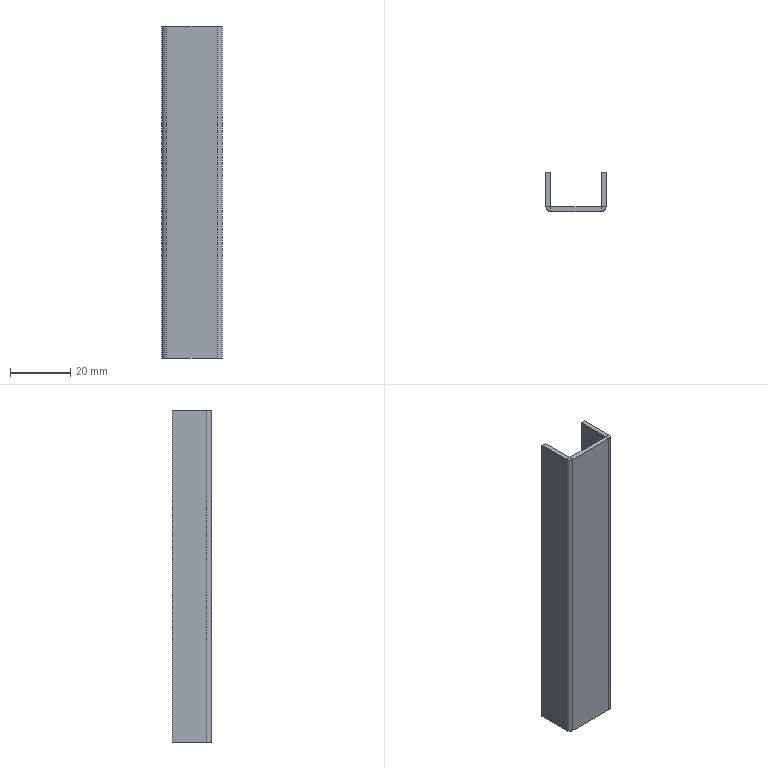Component | SolidWorks | P16BoxWeldment-1_BoxSupport-1 | 1 solid | 22 faces | box 20 x 13 x 110.6 mm | volume 7013 mm3 | plane 18 | cylinder 4 | commonest cylinder face diameters 3.2 x2 0.2 x2
STEP:
#1=COLOUR_RGB('',0.7922,0.8196,0.9333);
#2=FILL_AREA_STYLE_COLOUR('',#1);
#3=FILL_AREA_STYLE('',(#2));
#4=SURFACE_STYLE_FILL_AREA(#3);
#5=SURFACE_SIDE_STYLE('',(#4));
#6=SURFACE_STYLE_USAGE(.BOTH.,#5);
#7=PRESENTATION_STYLE_ASSIGNMENT((#6));
#8=CARTESIAN_POINT('',(-3.126,0.3402,2.409));
#9=VERTEX_POINT('',#8);
#10=CARTESIAN_POINT('',(-3.067,0.3402,2.409));
#11=VERTEX_POINT('',#10);
#12=CARTESIAN_POINT('',(-3.126,0.3402,2.409));
#13=DIRECTION('',(1.,0.,0.));
#14=VECTOR('',#13,39.37);
#15=LINE('',#12,#14);
#16=EDGE_CURVE('',#9,#11,#15,.T.);
#17=ORIENTED_EDGE('',*,*,#16,.F.);
#18=CARTESIAN_POINT('',(-3.063,0.2772,2.409));
#19=VERTEX_POINT('',#18);
#20=CARTESIAN_POINT('',(-3.063,0.3402,2.409));
#21=DIRECTION('',(0.,0.,-1.));
#22=DIRECTION('',(-1.,0.,0.));
#23=AXIS2_PLACEMENT_3D('',#20,#21,#22);
#24=CIRCLE('',#23,0.06299);
#25=EDGE_CURVE('',#19,#9,#24,.T.);
#26=ORIENTED_EDGE('',*,*,#25,.F.);
#27=CARTESIAN_POINT('',(-3.063,0.3363,2.409));
#28=VERTEX_POINT('',#27);
#29=CARTESIAN_POINT('',(-3.063,0.3363,2.409));
#30=DIRECTION('',(0.,-1.,0.));
#31=VECTOR('',#30,39.37);
#32=LINE('',#29,#31);
#33=EDGE_CURVE('',#28,#19,#32,.T.);
#34=ORIENTED_EDGE('',*,*,#33,.F.);
#35=CARTESIAN_POINT('',(-3.063,0.3402,2.409));
#36=DIRECTION('',(0.,0.,-1.));
#37=DIRECTION('',(1.,0.,0.));
#38=AXIS2_PLACEMENT_3D('',#35,#36,#37);
#39=CIRCLE('',#38,0.003937);
#40=EDGE_CURVE('',#28,#11,#39,.T.);
#41=ORIENTED_EDGE('',*,*,#40,.T.);
#42=EDGE_LOOP('',(#17,#26,#34,#41));
#43=FACE_OUTER_BOUND('',#42,.T.);
#44=CARTESIAN_POINT('',(-3.126,0.3402,2.409));
#45=DIRECTION('',(0.,0.,1.));
#46=DIRECTION('',(1.,0.,0.));
#47=AXIS2_PLACEMENT_3D('',#44,#45,#46);
#48=PLANE('',#47);
#49=ADVANCED_FACE('',(#43),#48,.T.);
#50=CARTESIAN_POINT('',(-3.126,0.7891,2.409));
#51=VERTEX_POINT('',#50);
#52=CARTESIAN_POINT('',(-3.126,0.7891,2.409));
#53=DIRECTION('',(-0.,1.,0.));
#54=VECTOR('',#53,39.37);
#55=LINE('',#52,#54);
#56=EDGE_CURVE('',#9,#51,#55,.T.);
#57=ORIENTED_EDGE('',*,*,#56,.F.);
#58=ORIENTED_EDGE('',*,*,#16,.T.);
#59=CARTESIAN_POINT('',(-3.067,0.7891,2.409));
#60=VERTEX_POINT('',#59);
#61=CARTESIAN_POINT('',(-3.067,0.7891,2.409));
#62=DIRECTION('',(-0.,1.,0.));
#63=VECTOR('',#62,39.37);
#64=LINE('',#61,#63);
#65=EDGE_CURVE('',#11,#60,#64,.T.);
#66=ORIENTED_EDGE('',*,*,#65,.T.);
#67=CARTESIAN_POINT('',(-3.126,0.7891,2.409));
#68=DIRECTION('',(1.,0.,0.));
#69=VECTOR('',#68,39.37);
#70=LINE('',#67,#69);
#71=EDGE_CURVE('',#51,#60,#70,.T.);
#72=ORIENTED_EDGE('',*,*,#71,.F.);
#73=EDGE_LOOP('',(#57,#58,#66,#72));
#74=FACE_OUTER_BOUND('',#73,.T.);
#75=CARTESIAN_POINT('',(-3.063,0.3363,2.409));
#76=DIRECTION('',(0.,0.,1.));
#77=DIRECTION('',(1.,0.,0.));
#78=AXIS2_PLACEMENT_3D('',#75,#76,#77);
#79=PLANE('',#78);
#80=ADVANCED_FACE('',(#74),#79,.T.);
#81=CARTESIAN_POINT('',(-3.063,0.2772,-1.945));
#82=VERTEX_POINT('',#81);
#83=CARTESIAN_POINT('',(-3.063,0.3363,-1.945));
#84=VERTEX_POINT('',#83);
#85=CARTESIAN_POINT('',(-3.063,0.2772,-1.945));
#86=DIRECTION('',(0.,1.,0.));
#87=VECTOR('',#86,39.37);
#88=LINE('',#85,#87);
#89=EDGE_CURVE('',#82,#84,#88,.T.);
#90=ORIENTED_EDGE('',*,*,#89,.F.);
#91=CARTESIAN_POINT('',(-3.126,0.3402,-1.945));
#92=VERTEX_POINT('',#91);
#93=CARTESIAN_POINT('',(-3.063,0.3402,-1.945));
#94=DIRECTION('',(0.,0.,-1.));
#95=DIRECTION('',(-1.,0.,0.));
#96=AXIS2_PLACEMENT_3D('',#93,#94,#95);
#97=CIRCLE('',#96,0.06299);
#98=EDGE_CURVE('',#82,#92,#97,.T.);
#99=ORIENTED_EDGE('',*,*,#98,.T.);
#100=CARTESIAN_POINT('',(-3.067,0.3402,-1.945));
#101=VERTEX_POINT('',#100);
#102=CARTESIAN_POINT('',(-3.067,0.3402,-1.945));
#103=DIRECTION('',(-1.,0.,0.));
#104=VECTOR('',#103,39.37);
#105=LINE('',#102,#104);
#106=EDGE_CURVE('',#101,#92,#105,.T.);
#107=ORIENTED_EDGE('',*,*,#106,.F.);
#108=CARTESIAN_POINT('',(-3.063,0.3402,-1.945));
#109=DIRECTION('',(0.,0.,-1.));
#110=DIRECTION('',(1.,0.,0.));
#111=AXIS2_PLACEMENT_3D('',#108,#109,#110);
#112=CIRCLE('',#111,0.003937);
#113=EDGE_CURVE('',#84,#101,#112,.T.);
#114=ORIENTED_EDGE('',*,*,#113,.F.);
#115=EDGE_LOOP('',(#90,#99,#107,#114));
#116=FACE_OUTER_BOUND('',#115,.T.);
#117=CARTESIAN_POINT('',(-3.063,0.2772,-1.945));
#118=DIRECTION('',(0.,0.,-1.));
#119=DIRECTION('',(-1.,0.,0.));
#120=AXIS2_PLACEMENT_3D('',#117,#118,#119);
#121=PLANE('',#120);
#122=ADVANCED_FACE('',(#116),#121,.T.);
#123=CARTESIAN_POINT('',(-2.401,0.2772,-1.945));
#124=VERTEX_POINT('',#123);
#125=CARTESIAN_POINT('',(-3.126,0.2772,-1.945));
#126=DIRECTION('',(-1.,-0.,0.));
#127=VECTOR('',#126,39.37);
#128=LINE('',#125,#127);
#129=EDGE_CURVE('',#124,#82,#128,.T.);
#130=ORIENTED_EDGE('',*,*,#129,.T.);
#131=ORIENTED_EDGE('',*,*,#89,.T.);
#132=CARTESIAN_POINT('',(-2.401,0.3363,-1.945));
#133=VERTEX_POINT('',#132);
#134=CARTESIAN_POINT('',(-3.126,0.3363,-1.945));
#135=DIRECTION('',(-1.,-0.,0.));
#136=VECTOR('',#135,39.37);
#137=LINE('',#134,#136);
#138=EDGE_CURVE('',#133,#84,#137,.T.);
#139=ORIENTED_EDGE('',*,*,#138,.F.);
#140=CARTESIAN_POINT('',(-2.401,0.3363,-1.945));
#141=DIRECTION('',(0.,-1.,0.));
#142=VECTOR('',#141,39.37);
#143=LINE('',#140,#142);
#144=EDGE_CURVE('',#133,#124,#143,.T.);
#145=ORIENTED_EDGE('',*,*,#144,.T.);
#146=EDGE_LOOP('',(#130,#131,#139,#145));
#147=FACE_OUTER_BOUND('',#146,.T.);
#148=CARTESIAN_POINT('',(-3.067,0.3402,-1.945));
#149=DIRECTION('',(0.,0.,-1.));
#150=DIRECTION('',(-1.,0.,0.));
#151=AXIS2_PLACEMENT_3D('',#148,#149,#150);
#152=PLANE('',#151);
#153=ADVANCED_FACE('',(#147),#152,.T.);
#154=CARTESIAN_POINT('',(-2.401,0.2772,2.409));
#155=VERTEX_POINT('',#154);
#156=CARTESIAN_POINT('',(-2.401,0.3363,2.409));
#157=VERTEX_POINT('',#156);
#158=CARTESIAN_POINT('',(-2.401,0.2772,2.409));
#159=DIRECTION('',(0.,1.,0.));
#160=VECTOR('',#159,39.37);
#161=LINE('',#158,#160);
#162=EDGE_CURVE('',#155,#157,#161,.T.);
#163=ORIENTED_EDGE('',*,*,#162,.F.);
#164=CARTESIAN_POINT('',(-2.338,0.3402,2.409));
#165=VERTEX_POINT('',#164);
#166=CARTESIAN_POINT('',(-2.401,0.3402,2.409));
#167=DIRECTION('',(0.,0.,-1.));
#168=DIRECTION('',(-1.,0.,0.));
#169=AXIS2_PLACEMENT_3D('',#166,#167,#168);
#170=CIRCLE('',#169,0.06299);
#171=EDGE_CURVE('',#165,#155,#170,.T.);
#172=ORIENTED_EDGE('',*,*,#171,.F.);
#173=CARTESIAN_POINT('',(-2.397,0.3402,2.409));
#174=VERTEX_POINT('',#173);
#175=CARTESIAN_POINT('',(-2.397,0.3402,2.409));
#176=DIRECTION('',(1.,0.,0.));
#177=VECTOR('',#176,39.37);
#178=LINE('',#175,#177);
#179=EDGE_CURVE('',#174,#165,#178,.T.);
#180=ORIENTED_EDGE('',*,*,#179,.F.);
#181=CARTESIAN_POINT('',(-2.401,0.3402,2.409));
#182=DIRECTION('',(0.,0.,-1.));
#183=DIRECTION('',(1.,0.,0.));
#184=AXIS2_PLACEMENT_3D('',#181,#182,#183);
#185=CIRCLE('',#184,0.003937);
#186=EDGE_CURVE('',#174,#157,#185,.T.);
#187=ORIENTED_EDGE('',*,*,#186,.T.);
#188=EDGE_LOOP('',(#163,#172,#180,#187));
#189=FACE_OUTER_BOUND('',#188,.T.);
#190=CARTESIAN_POINT('',(-2.401,0.2772,2.409));
#191=DIRECTION('',(0.,0.,1.));
#192=DIRECTION('',(1.,0.,0.));
#193=AXIS2_PLACEMENT_3D('',#190,#191,#192);
#194=PLANE('',#193);
#195=ADVANCED_FACE('',(#189),#194,.T.);
#196=CARTESIAN_POINT('',(-3.126,0.2772,2.409));
#197=DIRECTION('',(-1.,-0.,0.));
#198=VECTOR('',#197,39.37);
#199=LINE('',#196,#198);
#200=EDGE_CURVE('',#155,#19,#199,.T.);
#201=ORIENTED_EDGE('',*,*,#200,.F.);
#202=ORIENTED_EDGE('',*,*,#162,.T.);
#203=CARTESIAN_POINT('',(-3.126,0.3363,2.409));
#204=DIRECTION('',(-1.,-0.,0.));
#205=VECTOR('',#204,39.37);
#206=LINE('',#203,#205);
#207=EDGE_CURVE('',#157,#28,#206,.T.);
#208=ORIENTED_EDGE('',*,*,#207,.T.);
#209=ORIENTED_EDGE('',*,*,#33,.T.);
#210=EDGE_LOOP('',(#201,#202,#208,#209));
#211=FACE_OUTER_BOUND('',#210,.T.);
#212=CARTESIAN_POINT('',(-2.397,0.3402,2.409));
#213=DIRECTION('',(0.,0.,1.));
#214=DIRECTION('',(1.,0.,0.));
#215=AXIS2_PLACEMENT_3D('',#212,#213,#214);
#216=PLANE('',#215);
#217=ADVANCED_FACE('',(#211),#216,.T.);
#218=CARTESIAN_POINT('',(-2.338,0.3402,-1.945));
#219=VERTEX_POINT('',#218);
#220=CARTESIAN_POINT('',(-2.397,0.3402,-1.945));
#221=VERTEX_POINT('',#220);
#222=CARTESIAN_POINT('',(-2.338,0.3402,-1.945));
#223=DIRECTION('',(-1.,-0.,0.));
#224=VECTOR('',#223,39.37);
#225=LINE('',#222,#224);
#226=EDGE_CURVE('',#219,#221,#225,.T.);
#227=ORIENTED_EDGE('',*,*,#226,.F.);
#228=CARTESIAN_POINT('',(-2.401,0.3402,-1.945));
#229=DIRECTION('',(0.,0.,-1.));
#230=DIRECTION('',(-1.,0.,0.));
#231=AXIS2_PLACEMENT_3D('',#228,#229,#230);
#232=CIRCLE('',#231,0.06299);
#233=EDGE_CURVE('',#219,#124,#232,.T.);
#234=ORIENTED_EDGE('',*,*,#233,.T.);
#235=ORIENTED_EDGE('',*,*,#144,.F.);
#236=CARTESIAN_POINT('',(-2.401,0.3402,-1.945));
#237=DIRECTION('',(0.,0.,-1.));
#238=DIRECTION('',(1.,0.,0.));
#239=AXIS2_PLACEMENT_3D('',#236,#237,#238);
#240=CIRCLE('',#239,0.003937);
#241=EDGE_CURVE('',#221,#133,#240,.T.);
#242=ORIENTED_EDGE('',*,*,#241,.F.);
#243=EDGE_LOOP('',(#227,#234,#235,#242));
#244=FACE_OUTER_BOUND('',#243,.T.);
#245=CARTESIAN_POINT('',(-2.338,0.3402,-1.945));
#246=DIRECTION('',(0.,0.,-1.));
#247=DIRECTION('',(-1.,0.,0.));
#248=AXIS2_PLACEMENT_3D('',#245,#246,#247);
#249=PLANE('',#248);
#250=ADVANCED_FACE('',(#244),#249,.T.);
#251=CARTESIAN_POINT('',(-2.338,0.7891,-1.945));
#252=VERTEX_POINT('',#251);
#253=CARTESIAN_POINT('',(-2.338,0.7891,-1.945));
#254=DIRECTION('',(0.,-1.,0.));
#255=VECTOR('',#254,39.37);
#256=LINE('',#253,#255);
#257=EDGE_CURVE('',#252,#219,#256,.T.);
#258=ORIENTED_EDGE('',*,*,#257,.T.);
#259=ORIENTED_EDGE('',*,*,#226,.T.);
#260=CARTESIAN_POINT('',(-2.397,0.7891,-1.945));
#261=VERTEX_POINT('',#260);
#262=CARTESIAN_POINT('',(-2.397,0.7891,-1.945));
#263=DIRECTION('',(0.,-1.,0.));
#264=VECTOR('',#263,39.37);
#265=LINE('',#262,#264);
#266=EDGE_CURVE('',#261,#221,#265,.T.);
#267=ORIENTED_EDGE('',*,*,#266,.F.);
#268=CARTESIAN_POINT('',(-2.397,0.7891,-1.945));
#269=DIRECTION('',(1.,0.,0.));
#270=VECTOR('',#269,39.37);
#271=LINE('',#268,#270);
#272=EDGE_CURVE('',#261,#252,#271,.T.);
#273=ORIENTED_EDGE('',*,*,#272,.T.);
#274=EDGE_LOOP('',(#258,#259,#267,#273));
#275=FACE_OUTER_BOUND('',#274,.T.);
#276=CARTESIAN_POINT('',(-2.401,0.3363,-1.945));
#277=DIRECTION('',(0.,0.,-1.));
#278=DIRECTION('',(-1.,0.,0.));
#279=AXIS2_PLACEMENT_3D('',#276,#277,#278);
#280=PLANE('',#279);
#281=ADVANCED_FACE('',(#275),#280,.T.);
#282=CARTESIAN_POINT('',(-3.067,0.7891,-1.945));
#283=VERTEX_POINT('',#282);
#284=CARTESIAN_POINT('',(-3.067,0.7891,-1.945));
#285=DIRECTION('',(-0.,1.,0.));
#286=VECTOR('',#285,39.37);
#287=LINE('',#284,#286);
#288=EDGE_CURVE('',#101,#283,#287,.T.);
#289=ORIENTED_EDGE('',*,*,#288,.T.);
#290=CARTESIAN_POINT('',(-3.067,0.7891,2.409));
#291=DIRECTION('',(0.,0.,-1.));
#292=VECTOR('',#291,39.37);
#293=LINE('',#290,#292);
#294=EDGE_CURVE('',#60,#283,#293,.T.);
#295=ORIENTED_EDGE('',*,*,#294,.F.);
#296=ORIENTED_EDGE('',*,*,#65,.F.);
#297=CARTESIAN_POINT('',(-3.067,0.3402,2.409));
#298=DIRECTION('',(0.,0.,-1.));
#299=VECTOR('',#298,39.37);
#300=LINE('',#297,#299);
#301=EDGE_CURVE('',#11,#101,#300,.T.);
#302=ORIENTED_EDGE('',*,*,#301,.T.);
#303=EDGE_LOOP('',(#289,#295,#296,#302));
#304=FACE_OUTER_BOUND('',#303,.T.);
#305=CARTESIAN_POINT('',(-3.067,0.7891,2.409));
#306=DIRECTION('',(-1.,-0.,0.));
#307=DIRECTION('',(0.,-1.,0.));
#308=AXIS2_PLACEMENT_3D('',#305,#306,#307);
#309=PLANE('',#308);
#310=ADVANCED_FACE('',(#304),#309,.F.);
#311=CARTESIAN_POINT('',(-3.126,0.7891,-1.945));
#312=VERTEX_POINT('',#311);
#313=CARTESIAN_POINT('',(-3.126,0.7891,-1.945));
#314=DIRECTION('',(1.,0.,0.));
#315=VECTOR('',#314,39.37);
#316=LINE('',#313,#315);
#317=EDGE_CURVE('',#312,#283,#316,.T.);
#318=ORIENTED_EDGE('',*,*,#317,.F.);
#319=CARTESIAN_POINT('',(-3.126,0.7891,2.409));
#320=DIRECTION('',(0.,0.,-1.));
#321=VECTOR('',#320,39.37);
#322=LINE('',#319,#321);
#323=EDGE_CURVE('',#51,#312,#322,.T.);
#324=ORIENTED_EDGE('',*,*,#323,.F.);
#325=ORIENTED_EDGE('',*,*,#71,.T.);
#326=ORIENTED_EDGE('',*,*,#294,.T.);
#327=EDGE_LOOP('',(#318,#324,#325,#326));
#328=FACE_OUTER_BOUND('',#327,.T.);
#329=CARTESIAN_POINT('',(-3.126,0.7891,2.409));
#330=DIRECTION('',(0.,1.,0.));
#331=DIRECTION('',(0.,0.,1.));
#332=AXIS2_PLACEMENT_3D('',#329,#330,#331);
#333=PLANE('',#332);
#334=ADVANCED_FACE('',(#328),#333,.T.);
#335=CARTESIAN_POINT('',(-3.126,0.7891,-1.945));
#336=DIRECTION('',(-0.,1.,0.));
#337=VECTOR('',#336,39.37);
#338=LINE('',#335,#337);
#339=EDGE_CURVE('',#92,#312,#338,.T.);
#340=ORIENTED_EDGE('',*,*,#339,.F.);
#341=CARTESIAN_POINT('',(-3.126,0.3402,2.409));
#342=DIRECTION('',(0.,0.,-1.));
#343=VECTOR('',#342,39.37);
#344=LINE('',#341,#343);
#345=EDGE_CURVE('',#9,#92,#344,.T.);
#346=ORIENTED_EDGE('',*,*,#345,.F.);
#347=ORIENTED_EDGE('',*,*,#56,.T.);
#348=ORIENTED_EDGE('',*,*,#323,.T.);
#349=EDGE_LOOP('',(#340,#346,#347,#348));
#350=FACE_OUTER_BOUND('',#349,.T.);
#351=CARTESIAN_POINT('',(-3.126,0.7891,2.409));
#352=DIRECTION('',(-1.,-0.,0.));
#353=DIRECTION('',(0.,-1.,0.));
#354=AXIS2_PLACEMENT_3D('',#351,#352,#353);
#355=PLANE('',#354);
#356=ADVANCED_FACE('',(#350),#355,.T.);
#357=ORIENTED_EDGE('',*,*,#98,.F.);
#358=CARTESIAN_POINT('',(-3.063,0.2772,2.409));
#359=DIRECTION('',(0.,0.,-1.));
#360=VECTOR('',#359,39.37);
#361=LINE('',#358,#360);
#362=EDGE_CURVE('',#19,#82,#361,.T.);
#363=ORIENTED_EDGE('',*,*,#362,.F.);
#364=ORIENTED_EDGE('',*,*,#25,.T.);
#365=ORIENTED_EDGE('',*,*,#345,.T.);
#366=EDGE_LOOP('',(#357,#363,#364,#365));
#367=FACE_OUTER_BOUND('',#366,.T.);
#368=CARTESIAN_POINT('',(-3.063,0.3402,2.409));
#369=DIRECTION('',(0.,0.,-1.));
#370=DIRECTION('',(-1.,0.,0.));
#371=AXIS2_PLACEMENT_3D('',#368,#369,#370);
#372=CYLINDRICAL_SURFACE('',#371,0.06299);
#373=ADVANCED_FACE('',(#367),#372,.T.);
#374=ORIENTED_EDGE('',*,*,#129,.F.);
#375=CARTESIAN_POINT('',(-2.401,0.2772,2.409));
#376=DIRECTION('',(0.,0.,-1.));
#377=VECTOR('',#376,39.37);
#378=LINE('',#375,#377);
#379=EDGE_CURVE('',#155,#124,#378,.T.);
#380=ORIENTED_EDGE('',*,*,#379,.F.);
#381=ORIENTED_EDGE('',*,*,#200,.T.);
#382=ORIENTED_EDGE('',*,*,#362,.T.);
#383=EDGE_LOOP('',(#374,#380,#381,#382));
#384=FACE_OUTER_BOUND('',#383,.T.);
#385=CARTESIAN_POINT('',(-3.126,0.2772,2.409));
#386=DIRECTION('',(0.,-1.,0.));
#387=DIRECTION('',(1.,0.,0.));
#388=AXIS2_PLACEMENT_3D('',#385,#386,#387);
#389=PLANE('',#388);
#390=ADVANCED_FACE('',(#384),#389,.T.);
#391=ORIENTED_EDGE('',*,*,#233,.F.);
#392=CARTESIAN_POINT('',(-2.338,0.3402,2.409));
#393=DIRECTION('',(0.,0.,-1.));
#394=VECTOR('',#393,39.37);
#395=LINE('',#392,#394);
#396=EDGE_CURVE('',#165,#219,#395,.T.);
#397=ORIENTED_EDGE('',*,*,#396,.F.);
#398=ORIENTED_EDGE('',*,*,#171,.T.);
#399=ORIENTED_EDGE('',*,*,#379,.T.);
#400=EDGE_LOOP('',(#391,#397,#398,#399));
#401=FACE_OUTER_BOUND('',#400,.T.);
#402=CARTESIAN_POINT('',(-2.401,0.3402,2.409));
#403=DIRECTION('',(0.,0.,-1.));
#404=DIRECTION('',(-1.,0.,0.));
#405=AXIS2_PLACEMENT_3D('',#402,#403,#404);
#406=CYLINDRICAL_SURFACE('',#405,0.06299);
#407=ADVANCED_FACE('',(#401),#406,.T.);
#408=ORIENTED_EDGE('',*,*,#257,.F.);
#409=CARTESIAN_POINT('',(-2.338,0.7891,2.409));
#410=VERTEX_POINT('',#409);
#411=CARTESIAN_POINT('',(-2.338,0.7891,2.409));
#412=DIRECTION('',(0.,0.,-1.));
#413=VECTOR('',#412,39.37);
#414=LINE('',#411,#413);
#415=EDGE_CURVE('',#410,#252,#414,.T.);
#416=ORIENTED_EDGE('',*,*,#415,.F.);
#417=CARTESIAN_POINT('',(-2.338,0.7891,2.409));
#418=DIRECTION('',(0.,-1.,0.));
#419=VECTOR('',#418,39.37);
#420=LINE('',#417,#419);
#421=EDGE_CURVE('',#410,#165,#420,.T.);
#422=ORIENTED_EDGE('',*,*,#421,.T.);
#423=ORIENTED_EDGE('',*,*,#396,.T.);
#424=EDGE_LOOP('',(#408,#416,#422,#423));
#425=FACE_OUTER_BOUND('',#424,.T.);
#426=CARTESIAN_POINT('',(-2.338,0.7891,2.409));
#427=DIRECTION('',(1.,0.,0.));
#428=DIRECTION('',(-0.,1.,0.));
#429=AXIS2_PLACEMENT_3D('',#426,#427,#428);
#430=PLANE('',#429);
#431=ADVANCED_FACE('',(#425),#430,.T.);
#432=ORIENTED_EDGE('',*,*,#272,.F.);
#433=CARTESIAN_POINT('',(-2.397,0.7891,2.409));
#434=VERTEX_POINT('',#433);
#435=CARTESIAN_POINT('',(-2.397,0.7891,2.409));
#436=DIRECTION('',(0.,0.,-1.));
#437=VECTOR('',#436,39.37);
#438=LINE('',#435,#437);
#439=EDGE_CURVE('',#434,#261,#438,.T.);
#440=ORIENTED_EDGE('',*,*,#439,.F.);
#441=CARTESIAN_POINT('',(-2.397,0.7891,2.409));
#442=DIRECTION('',(1.,0.,0.));
#443=VECTOR('',#442,39.37);
#444=LINE('',#441,#443);
#445=EDGE_CURVE('',#434,#410,#444,.T.);
#446=ORIENTED_EDGE('',*,*,#445,.T.);
#447=ORIENTED_EDGE('',*,*,#415,.T.);
#448=EDGE_LOOP('',(#432,#440,#446,#447));
#449=FACE_OUTER_BOUND('',#448,.T.);
#450=CARTESIAN_POINT('',(-2.397,0.7891,2.409));
#451=DIRECTION('',(0.,1.,0.));
#452=DIRECTION('',(0.,0.,1.));
#453=AXIS2_PLACEMENT_3D('',#450,#451,#452);
#454=PLANE('',#453);
#455=ADVANCED_FACE('',(#449),#454,.T.);
#456=ORIENTED_EDGE('',*,*,#266,.T.);
#457=CARTESIAN_POINT('',(-2.397,0.3402,2.409));
#458=DIRECTION('',(0.,0.,-1.));
#459=VECTOR('',#458,39.37);
#460=LINE('',#457,#459);
#461=EDGE_CURVE('',#174,#221,#460,.T.);
#462=ORIENTED_EDGE('',*,*,#461,.F.);
#463=CARTESIAN_POINT('',(-2.397,0.7891,2.409));
#464=DIRECTION('',(0.,-1.,0.));
#465=VECTOR('',#464,39.37);
#466=LINE('',#463,#465);
#467=EDGE_CURVE('',#434,#174,#466,.T.);
#468=ORIENTED_EDGE('',*,*,#467,.F.);
#469=ORIENTED_EDGE('',*,*,#439,.T.);
#470=EDGE_LOOP('',(#456,#462,#468,#469));
#471=FACE_OUTER_BOUND('',#470,.T.);
#472=CARTESIAN_POINT('',(-2.397,0.7891,2.409));
#473=DIRECTION('',(1.,0.,0.));
#474=DIRECTION('',(-0.,1.,0.));
#475=AXIS2_PLACEMENT_3D('',#472,#473,#474);
#476=PLANE('',#475);
#477=ADVANCED_FACE('',(#471),#476,.F.);
#478=ORIENTED_EDGE('',*,*,#241,.T.);
#479=CARTESIAN_POINT('',(-2.401,0.3363,2.409));
#480=DIRECTION('',(0.,0.,-1.));
#481=VECTOR('',#480,39.37);
#482=LINE('',#479,#481);
#483=EDGE_CURVE('',#157,#133,#482,.T.);
#484=ORIENTED_EDGE('',*,*,#483,.F.);
#485=ORIENTED_EDGE('',*,*,#186,.F.);
#486=ORIENTED_EDGE('',*,*,#461,.T.);
#487=EDGE_LOOP('',(#478,#484,#485,#486));
#488=FACE_OUTER_BOUND('',#487,.T.);
#489=CARTESIAN_POINT('',(-2.401,0.3402,2.409));
#490=DIRECTION('',(0.,0.,-1.));
#491=DIRECTION('',(-1.,0.,0.));
#492=AXIS2_PLACEMENT_3D('',#489,#490,#491);
#493=CYLINDRICAL_SURFACE('',#492,0.003937);
#494=ADVANCED_FACE('',(#488),#493,.F.);
#495=ORIENTED_EDGE('',*,*,#138,.T.);
#496=CARTESIAN_POINT('',(-3.063,0.3363,2.409));
#497=DIRECTION('',(0.,0.,-1.));
#498=VECTOR('',#497,39.37);
#499=LINE('',#496,#498);
#500=EDGE_CURVE('',#28,#84,#499,.T.);
#501=ORIENTED_EDGE('',*,*,#500,.F.);
#502=ORIENTED_EDGE('',*,*,#207,.F.);
#503=ORIENTED_EDGE('',*,*,#483,.T.);
#504=EDGE_LOOP('',(#495,#501,#502,#503));
#505=FACE_OUTER_BOUND('',#504,.T.);
#506=CARTESIAN_POINT('',(-3.126,0.3363,2.409));
#507=DIRECTION('',(0.,-1.,0.));
#508=DIRECTION('',(1.,0.,0.));
#509=AXIS2_PLACEMENT_3D('',#506,#507,#508);
#510=PLANE('',#509);
#511=ADVANCED_FACE('',(#505),#510,.F.);
#512=ORIENTED_EDGE('',*,*,#113,.T.);
#513=ORIENTED_EDGE('',*,*,#301,.F.);
#514=ORIENTED_EDGE('',*,*,#40,.F.);
#515=ORIENTED_EDGE('',*,*,#500,.T.);
#516=EDGE_LOOP('',(#512,#513,#514,#515));
#517=FACE_OUTER_BOUND('',#516,.T.);
#518=CARTESIAN_POINT('',(-3.063,0.3402,2.409));
#519=DIRECTION('',(0.,0.,-1.));
#520=DIRECTION('',(-1.,0.,0.));
#521=AXIS2_PLACEMENT_3D('',#518,#519,#520);
#522=CYLINDRICAL_SURFACE('',#521,0.003937);
#523=ADVANCED_FACE('',(#517),#522,.F.);
#524=ORIENTED_EDGE('',*,*,#467,.T.);
#525=ORIENTED_EDGE('',*,*,#179,.T.);
#526=ORIENTED_EDGE('',*,*,#421,.F.);
#527=ORIENTED_EDGE('',*,*,#445,.F.);
#528=EDGE_LOOP('',(#524,#525,#526,#527));
#529=FACE_OUTER_BOUND('',#528,.T.);
#530=CARTESIAN_POINT('',(-3.063,0.3402,2.409));
#531=DIRECTION('',(0.,0.,-1.));
#532=DIRECTION('',(-1.,0.,0.));
#533=AXIS2_PLACEMENT_3D('',#530,#531,#532);
#534=PLANE('',#533);
#535=ADVANCED_FACE('',(#529),#534,.F.);
#536=ORIENTED_EDGE('',*,*,#288,.F.);
#537=ORIENTED_EDGE('',*,*,#106,.T.);
#538=ORIENTED_EDGE('',*,*,#339,.T.);
#539=ORIENTED_EDGE('',*,*,#317,.T.);
#540=EDGE_LOOP('',(#536,#537,#538,#539));
#541=FACE_OUTER_BOUND('',#540,.T.);
#542=CARTESIAN_POINT('',(-3.063,0.3402,-1.945));
#543=DIRECTION('',(0.,0.,-1.));
#544=DIRECTION('',(-1.,0.,0.));
#545=AXIS2_PLACEMENT_3D('',#542,#543,#544);
#546=PLANE('',#545);
#547=ADVANCED_FACE('',(#541),#546,.T.);
#548=CLOSED_SHELL('',(#49,#80,#122,#153,#195,#217,#250,#281,#310,#334,#356,#373,#390,#407,#431,#455,#477,#494,#511,#523,#535,#547));
#549=MANIFOLD_SOLID_BREP('',#548);
#550=STYLED_ITEM('',(#7),#549);
#551=(LENGTH_UNIT()NAMED_UNIT(*)SI_UNIT($,.METRE.));
#552=LENGTH_MEASURE_WITH_UNIT(LENGTH_MEASURE(0.0254),#551);
#553=DIMENSIONAL_EXPONENTS(1.,0.,0.,0.,0.,0.,0.);
#554=(CONVERSION_BASED_UNIT('',#552)LENGTH_UNIT()NAMED_UNIT(#553));
#555=UNCERTAINTY_MEASURE_WITH_UNIT(LENGTH_MEASURE(0.00001),#554,'','');
#556=(NAMED_UNIT(*)PLANE_ANGLE_UNIT()SI_UNIT($,.RADIAN.));
#557=(NAMED_UNIT(*)SI_UNIT($,.STERADIAN.)SOLID_ANGLE_UNIT());
#558=(GEOMETRIC_REPRESENTATION_CONTEXT(3)GLOBAL_UNCERTAINTY_ASSIGNED_CONTEXT((#555))GLOBAL_UNIT_ASSIGNED_CONTEXT((#554,#556,#557))REPRESENTATION_CONTEXT('',''));
#559=MECHANICAL_DESIGN_GEOMETRIC_PRESENTATION_REPRESENTATION('',(#550),#558);
#560=PRESENTATION_LAYER_ASSIGNMENT('','',(#550));
#561=CARTESIAN_POINT('',(0.,0.,0.));
#562=DIRECTION('',(0.,0.,1.));
#563=DIRECTION('',(1.,0.,0.));
#564=AXIS2_PLACEMENT_3D('',#561,#562,#563);
#565=(LENGTH_UNIT()NAMED_UNIT(*)SI_UNIT($,.METRE.));
#566=LENGTH_MEASURE_WITH_UNIT(LENGTH_MEASURE(0.0254),#565);
#567=DIMENSIONAL_EXPONENTS(1.,0.,0.,0.,0.,0.,0.);
#568=(CONVERSION_BASED_UNIT('',#566)LENGTH_UNIT()NAMED_UNIT(#567));
#569=UNCERTAINTY_MEASURE_WITH_UNIT(LENGTH_MEASURE(0.00001),#568,'','');
#570=(NAMED_UNIT(*)PLANE_ANGLE_UNIT()SI_UNIT($,.RADIAN.));
#571=(NAMED_UNIT(*)SI_UNIT($,.STERADIAN.)SOLID_ANGLE_UNIT());
#572=(GEOMETRIC_REPRESENTATION_CONTEXT(3)GLOBAL_UNCERTAINTY_ASSIGNED_CONTEXT((#569))GLOBAL_UNIT_ASSIGNED_CONTEXT((#568,#570,#571))REPRESENTATION_CONTEXT('',''));
#573=ADVANCED_BREP_SHAPE_REPRESENTATION('',(#549,#564),#572);